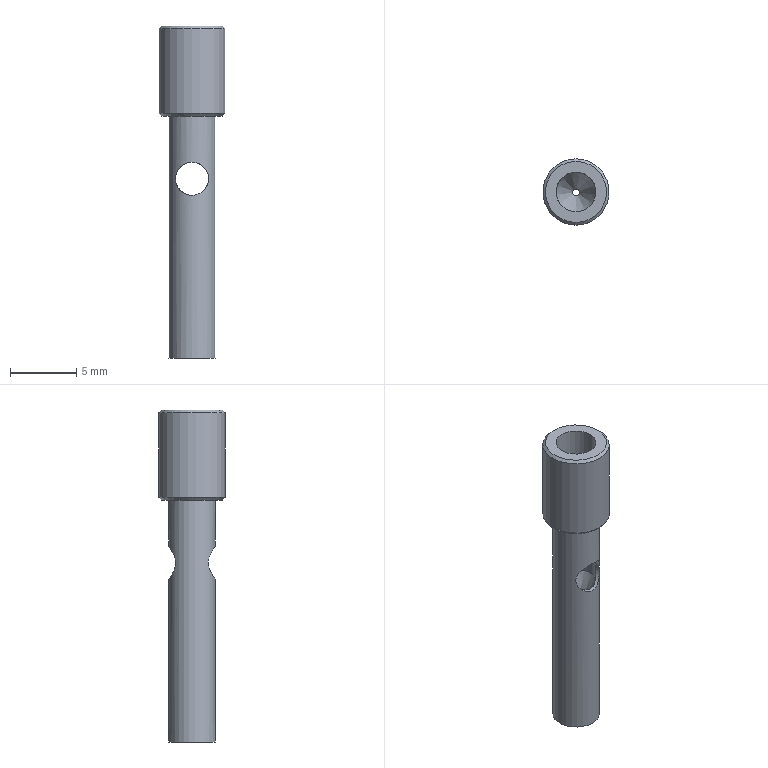Component | NX | AIR_PUMP_PART_01_11 | 1 solid | 14 faces | volume 187 mm3 | cylinder 7 | plane 4 | cone 3 | commonest cylinder face diameters 2.5 x3 3.5 x1 3 x1 5 x1 0.5 x1